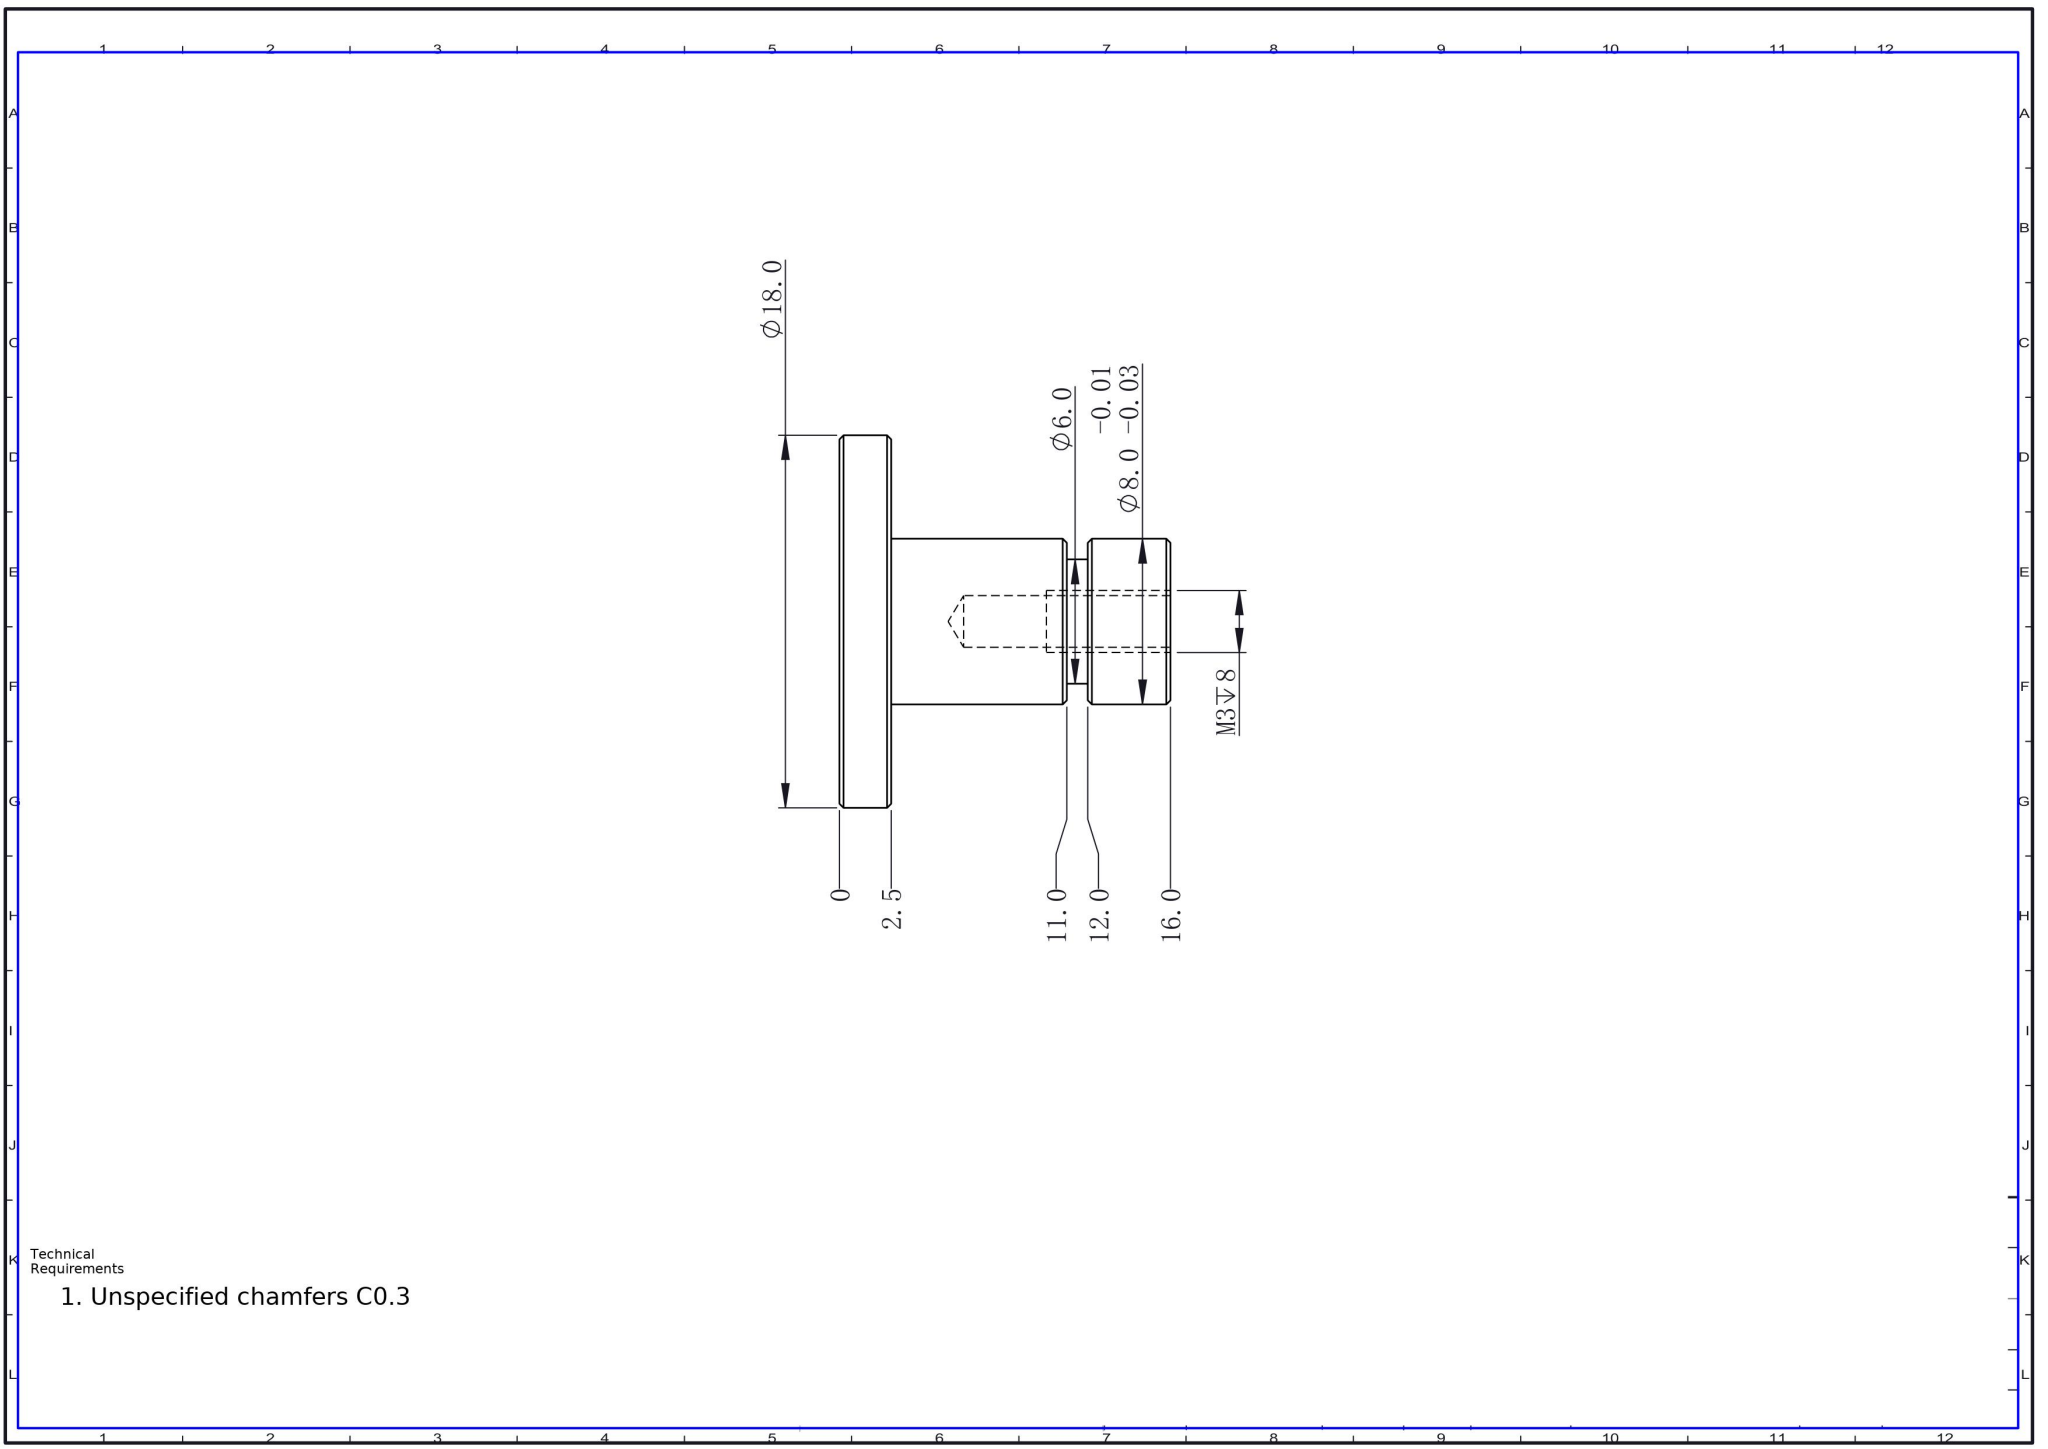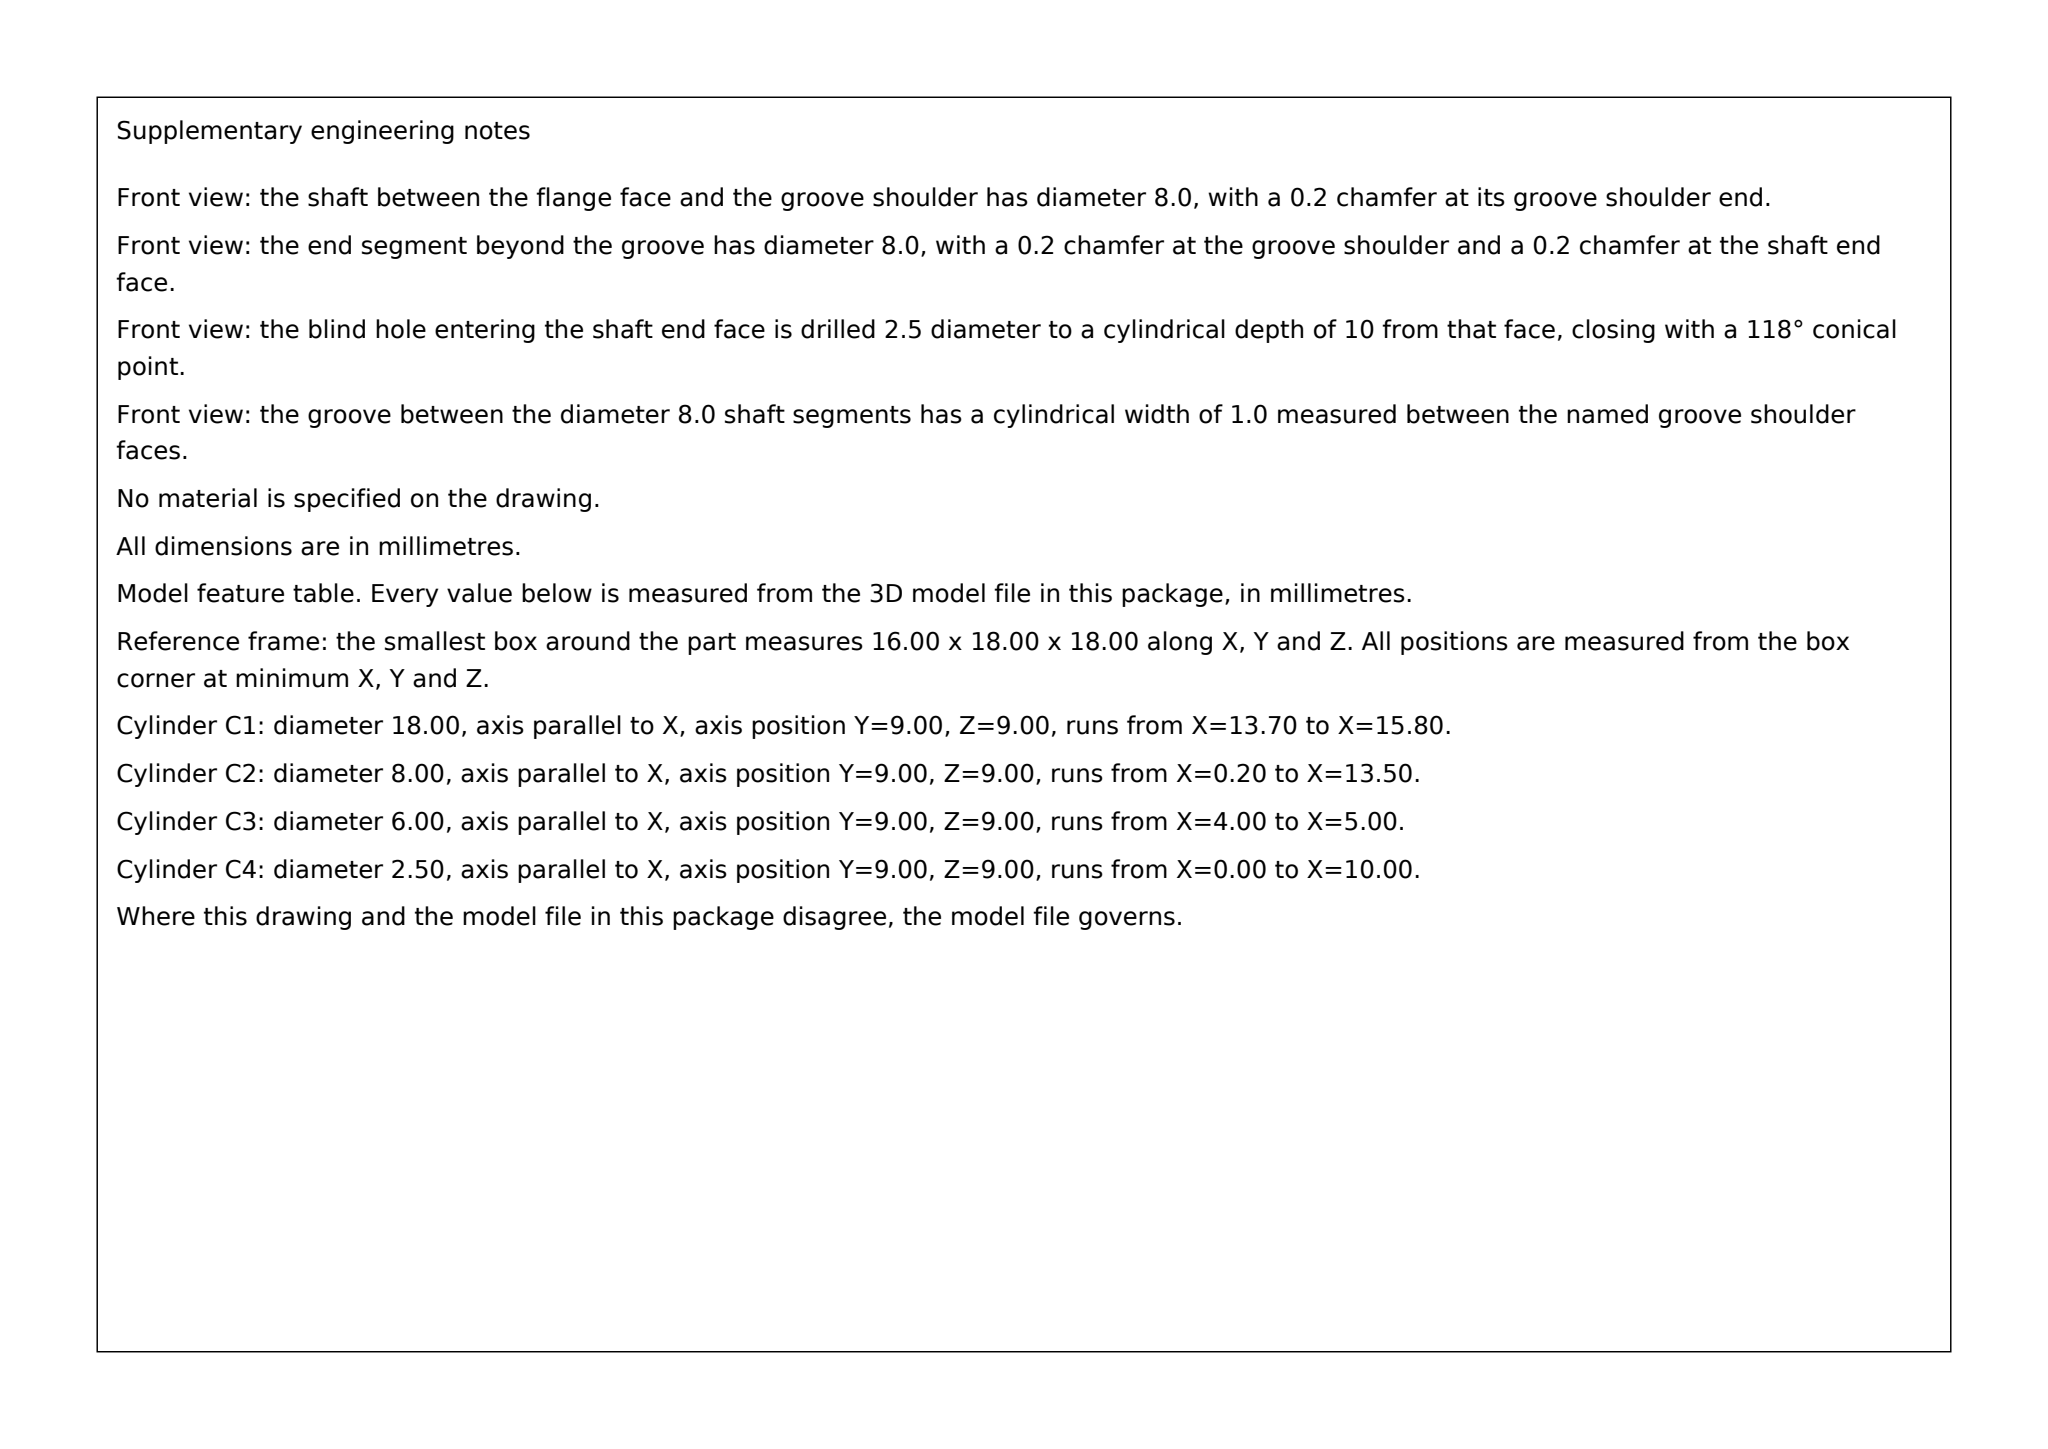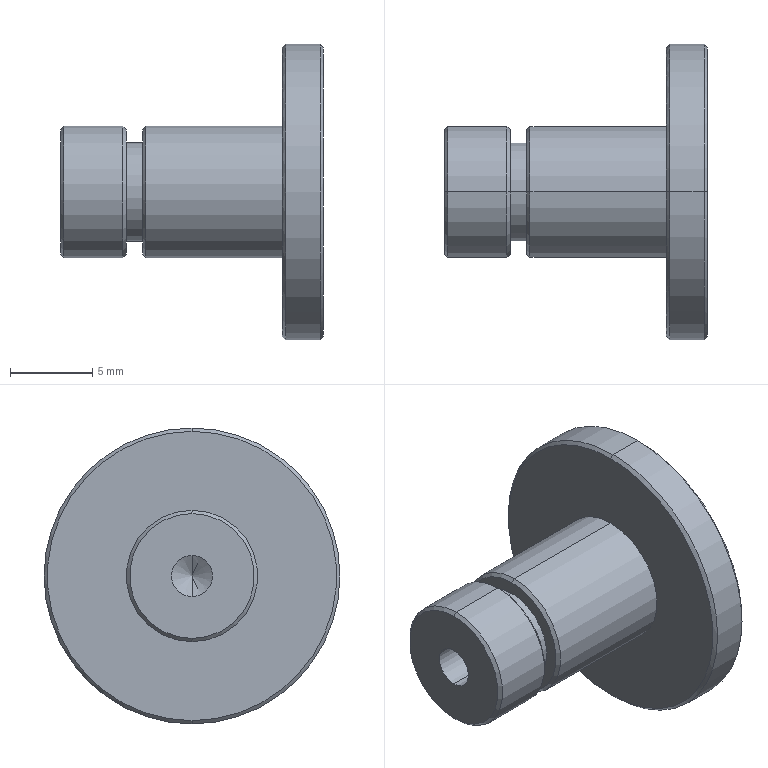Part | SolidWorks | mm | 1 solid | 27 faces | box 16 x 18 x 18 mm | volume 1239 mm3 | cone 12 | cylinder 10 | plane 5 | commonest cylinder face diameters 8 x4 2.5 x2 6 x2 18 x2
Drawing notes:
Ø8.0 SHAFT FROM FLANGE FACE (2.5) TO Ø6.0 GROOVE (11.0) | from the solid: cylinder dia 8.0, axis x, len 8.3 between 18.0 flange and 6.0 groove (2.5-11.0 nominal)
TAP DRILL Ø2.5 DP 10 FROM END FACE (16.0), 118° PT | from the solid: cylinder dia 2.5 axis x len 10.0 + cone 118° ref dia 2.5, open at x=16 end face
CHAMFER C0.2 x 45 ON BOTH Ø18 FLANGE OUTER EDGES (AT 0 AND 2.5 FROM FLANGE BACK FACE) | from the solid: cones[90.0,18.0] and cones[90.0,17.6]: (18.0-17.6)/2 = 0.2 chamfer leg at 45 deg on Ø18 cylinder (length 2.1, axis x)
CHAMFER C0.2 x 45 ON ALL Ø8 SHAFT AND BOSS END EDGES, INCL. END FACE AT 16.0 FROM FLANGE BACK FACE (0) | from the solid: cones[90.0,8.0] and cones[90.0,7.6] (4X): (8.0-7.6)/2 = 0.2 chamfer leg at 45 deg on Ø8 cylinders; x-planes at 13.5 and 16.0
STEP:
#1=CARTESIAN_POINT('',(9.,0.,-1.25));
#2=VERTEX_POINT('',#1);
#3=CARTESIAN_POINT('',(9.,0.,1.25));
#4=VERTEX_POINT('',#3);
#5=CARTESIAN_POINT('',(9.,0.,0.));
#6=DIRECTION('',(-1.,0.,0.));
#7=DIRECTION('',(0.,0.,1.));
#8=AXIS2_PLACEMENT_3D('',#5,#6,#7);
#9=CIRCLE('',#8,1.25);
#10=EDGE_CURVE('',#2,#4,#9,.T.);
#11=ORIENTED_EDGE('',*,*,#10,.F.);
#12=CARTESIAN_POINT('',(-1.,0.,-1.25));
#13=VERTEX_POINT('',#12);
#14=CARTESIAN_POINT('',(-1.,0.,-1.25));
#15=DIRECTION('',(-1.,0.,0.));
#16=VECTOR('',#15,1000.);
#17=LINE('',#14,#16);
#18=EDGE_CURVE('',#2,#13,#17,.T.);
#19=ORIENTED_EDGE('',*,*,#18,.T.);
#20=CARTESIAN_POINT('',(-1.,0.,1.25));
#21=VERTEX_POINT('',#20);
#22=CARTESIAN_POINT('',(-1.,0.,0.));
#23=DIRECTION('',(-1.,0.,0.));
#24=DIRECTION('',(0.,0.,1.));
#25=AXIS2_PLACEMENT_3D('',#22,#23,#24);
#26=CIRCLE('',#25,1.25);
#27=EDGE_CURVE('',#13,#21,#26,.T.);
#28=ORIENTED_EDGE('',*,*,#27,.T.);
#29=CARTESIAN_POINT('',(-1.,0.,1.25));
#30=DIRECTION('',(-1.,0.,0.));
#31=VECTOR('',#30,1000.);
#32=LINE('',#29,#31);
#33=EDGE_CURVE('',#4,#21,#32,.T.);
#34=ORIENTED_EDGE('',*,*,#33,.F.);
#35=EDGE_LOOP('',(#11,#19,#28,#34));
#36=FACE_OUTER_BOUND('',#35,.T.);
#37=CARTESIAN_POINT('',(-1.,0.,0.));
#38=DIRECTION('',(-1.,0.,0.));
#39=DIRECTION('',(0.,0.,1.));
#40=AXIS2_PLACEMENT_3D('',#37,#38,#39);
#41=CYLINDRICAL_SURFACE('',#40,1.25);
#42=ADVANCED_FACE('',(#36),#41,.F.);
#43=CARTESIAN_POINT('',(9.751,-0.,0.));
#44=VERTEX_POINT('',#43);
#45=CARTESIAN_POINT('',(9.,0.,1.25));
#46=DIRECTION('',(-0.515,0.,0.8572));
#47=VECTOR('',#46,1000.);
#48=LINE('',#45,#47);
#49=EDGE_CURVE('',#44,#4,#48,.T.);
#50=ORIENTED_EDGE('',*,*,#49,.F.);
#51=CARTESIAN_POINT('',(9.,0.,-1.25));
#52=DIRECTION('',(-0.515,0.,-0.8572));
#53=VECTOR('',#52,1000.);
#54=LINE('',#51,#53);
#55=EDGE_CURVE('',#44,#2,#54,.T.);
#56=ORIENTED_EDGE('',*,*,#55,.T.);
#57=ORIENTED_EDGE('',*,*,#10,.T.);
#58=EDGE_LOOP('',(#50,#56,#57));
#59=FACE_OUTER_BOUND('',#58,.T.);
#60=CARTESIAN_POINT('',(9.,0.,0.));
#61=DIRECTION('',(-1.,0.,0.));
#62=DIRECTION('',(0.,0.,1.));
#63=AXIS2_PLACEMENT_3D('',#60,#61,#62);
#64=CONICAL_SURFACE('',#63,1.25,1.03);
#65=ADVANCED_FACE('',(#59),#64,.F.);
#66=CARTESIAN_POINT('',(15.,0.,-8.8));
#67=VERTEX_POINT('',#66);
#68=CARTESIAN_POINT('',(15.,0.,8.8));
#69=VERTEX_POINT('',#68);
#70=CARTESIAN_POINT('',(15.,0.,0.));
#71=DIRECTION('',(1.,0.,0.));
#72=DIRECTION('',(0.,0.,1.));
#73=AXIS2_PLACEMENT_3D('',#70,#71,#72);
#74=CIRCLE('',#73,8.8);
#75=EDGE_CURVE('',#67,#69,#74,.T.);
#76=ORIENTED_EDGE('',*,*,#75,.F.);
#77=CARTESIAN_POINT('',(14.8,0.,-9.));
#78=VERTEX_POINT('',#77);
#79=CARTESIAN_POINT('',(14.8,0.,-9.));
#80=DIRECTION('',(-0.7071,0.,-0.7071));
#81=VECTOR('',#80,1000.);
#82=LINE('',#79,#81);
#83=EDGE_CURVE('',#67,#78,#82,.T.);
#84=ORIENTED_EDGE('',*,*,#83,.T.);
#85=CARTESIAN_POINT('',(14.8,0.,9.));
#86=VERTEX_POINT('',#85);
#87=CARTESIAN_POINT('',(14.8,0.,0.));
#88=DIRECTION('',(-1.,0.,0.));
#89=DIRECTION('',(0.,0.,1.));
#90=AXIS2_PLACEMENT_3D('',#87,#88,#89);
#91=CIRCLE('',#90,9.);
#92=EDGE_CURVE('',#86,#78,#91,.T.);
#93=ORIENTED_EDGE('',*,*,#92,.F.);
#94=CARTESIAN_POINT('',(14.8,0.,9.));
#95=DIRECTION('',(-0.7071,0.,0.7071));
#96=VECTOR('',#95,1000.);
#97=LINE('',#94,#96);
#98=EDGE_CURVE('',#69,#86,#97,.T.);
#99=ORIENTED_EDGE('',*,*,#98,.F.);
#100=EDGE_LOOP('',(#76,#84,#93,#99));
#101=FACE_OUTER_BOUND('',#100,.T.);
#102=CARTESIAN_POINT('',(14.8,0.,0.));
#103=DIRECTION('',(-1.,0.,0.));
#104=DIRECTION('',(0.,0.,1.));
#105=AXIS2_PLACEMENT_3D('',#102,#103,#104);
#106=CONICAL_SURFACE('',#105,9.,0.7854);
#107=ADVANCED_FACE('',(#101),#106,.T.);
#108=CARTESIAN_POINT('',(12.5,0.,8.8));
#109=VERTEX_POINT('',#108);
#110=CARTESIAN_POINT('',(12.5,0.,-8.8));
#111=VERTEX_POINT('',#110);
#112=CARTESIAN_POINT('',(12.5,0.,0.));
#113=DIRECTION('',(-1.,0.,0.));
#114=DIRECTION('',(0.,0.,-1.));
#115=AXIS2_PLACEMENT_3D('',#112,#113,#114);
#116=CIRCLE('',#115,8.8);
#117=EDGE_CURVE('',#109,#111,#116,.T.);
#118=ORIENTED_EDGE('',*,*,#117,.F.);
#119=CARTESIAN_POINT('',(12.7,0.,9.));
#120=VERTEX_POINT('',#119);
#121=CARTESIAN_POINT('',(12.5,0.,8.8));
#122=DIRECTION('',(0.7071,0.,0.7071));
#123=VECTOR('',#122,1000.);
#124=LINE('',#121,#123);
#125=EDGE_CURVE('',#109,#120,#124,.T.);
#126=ORIENTED_EDGE('',*,*,#125,.T.);
#127=CARTESIAN_POINT('',(12.7,0.,-9.));
#128=VERTEX_POINT('',#127);
#129=CARTESIAN_POINT('',(12.7,0.,0.));
#130=DIRECTION('',(1.,0.,0.));
#131=DIRECTION('',(0.,0.,-1.));
#132=AXIS2_PLACEMENT_3D('',#129,#130,#131);
#133=CIRCLE('',#132,9.);
#134=EDGE_CURVE('',#128,#120,#133,.T.);
#135=ORIENTED_EDGE('',*,*,#134,.F.);
#136=CARTESIAN_POINT('',(12.5,0.,-8.8));
#137=DIRECTION('',(0.7071,0.,-0.7071));
#138=VECTOR('',#137,1000.);
#139=LINE('',#136,#138);
#140=EDGE_CURVE('',#111,#128,#139,.T.);
#141=ORIENTED_EDGE('',*,*,#140,.F.);
#142=EDGE_LOOP('',(#118,#126,#135,#141));
#143=FACE_OUTER_BOUND('',#142,.T.);
#144=CARTESIAN_POINT('',(12.5,0.,0.));
#145=DIRECTION('',(1.,0.,0.));
#146=DIRECTION('',(0.,0.,-1.));
#147=AXIS2_PLACEMENT_3D('',#144,#145,#146);
#148=CONICAL_SURFACE('',#147,8.8,0.7854);
#149=ADVANCED_FACE('',(#143),#148,.T.);
#150=CARTESIAN_POINT('',(-1.,0.,3.8));
#151=VERTEX_POINT('',#150);
#152=CARTESIAN_POINT('',(-1.,0.,-3.8));
#153=VERTEX_POINT('',#152);
#154=CARTESIAN_POINT('',(-1.,0.,0.));
#155=DIRECTION('',(-1.,0.,0.));
#156=DIRECTION('',(0.,0.,-1.));
#157=AXIS2_PLACEMENT_3D('',#154,#155,#156);
#158=CIRCLE('',#157,3.8);
#159=EDGE_CURVE('',#151,#153,#158,.T.);
#160=ORIENTED_EDGE('',*,*,#159,.F.);
#161=CARTESIAN_POINT('',(-0.8,0.,4.));
#162=VERTEX_POINT('',#161);
#163=CARTESIAN_POINT('',(-1.,0.,3.8));
#164=DIRECTION('',(0.7071,0.,0.7071));
#165=VECTOR('',#164,1000.);
#166=LINE('',#163,#165);
#167=EDGE_CURVE('',#151,#162,#166,.T.);
#168=ORIENTED_EDGE('',*,*,#167,.T.);
#169=CARTESIAN_POINT('',(-0.8,0.,-4.));
#170=VERTEX_POINT('',#169);
#171=CARTESIAN_POINT('',(-0.8,0.,0.));
#172=DIRECTION('',(1.,0.,0.));
#173=DIRECTION('',(0.,0.,-1.));
#174=AXIS2_PLACEMENT_3D('',#171,#172,#173);
#175=CIRCLE('',#174,4.);
#176=EDGE_CURVE('',#170,#162,#175,.T.);
#177=ORIENTED_EDGE('',*,*,#176,.F.);
#178=CARTESIAN_POINT('',(-1.,0.,-3.8));
#179=DIRECTION('',(0.7071,0.,-0.7071));
#180=VECTOR('',#179,1000.);
#181=LINE('',#178,#180);
#182=EDGE_CURVE('',#153,#170,#181,.T.);
#183=ORIENTED_EDGE('',*,*,#182,.F.);
#184=EDGE_LOOP('',(#160,#168,#177,#183));
#185=FACE_OUTER_BOUND('',#184,.T.);
#186=CARTESIAN_POINT('',(-1.,0.,0.));
#187=DIRECTION('',(1.,0.,0.));
#188=DIRECTION('',(0.,0.,-1.));
#189=AXIS2_PLACEMENT_3D('',#186,#187,#188);
#190=CONICAL_SURFACE('',#189,3.8,0.7854);
#191=ADVANCED_FACE('',(#185),#190,.T.);
#192=CARTESIAN_POINT('',(4.,0.,3.8));
#193=VERTEX_POINT('',#192);
#194=CARTESIAN_POINT('',(4.,0.,-3.8));
#195=VERTEX_POINT('',#194);
#196=CARTESIAN_POINT('',(4.,0.,0.));
#197=DIRECTION('',(-1.,0.,0.));
#198=DIRECTION('',(0.,0.,1.));
#199=AXIS2_PLACEMENT_3D('',#196,#197,#198);
#200=CIRCLE('',#199,3.8);
#201=EDGE_CURVE('',#193,#195,#200,.T.);
#202=ORIENTED_EDGE('',*,*,#201,.F.);
#203=CARTESIAN_POINT('',(4.2,0.,4.));
#204=VERTEX_POINT('',#203);
#205=CARTESIAN_POINT('',(4.,0.,3.8));
#206=DIRECTION('',(0.7071,0.,0.7071));
#207=VECTOR('',#206,1000.);
#208=LINE('',#205,#207);
#209=EDGE_CURVE('',#193,#204,#208,.T.);
#210=ORIENTED_EDGE('',*,*,#209,.T.);
#211=CARTESIAN_POINT('',(4.2,0.,-4.));
#212=VERTEX_POINT('',#211);
#213=CARTESIAN_POINT('',(4.2,0.,0.));
#214=DIRECTION('',(1.,0.,0.));
#215=DIRECTION('',(0.,0.,1.));
#216=AXIS2_PLACEMENT_3D('',#213,#214,#215);
#217=CIRCLE('',#216,4.);
#218=EDGE_CURVE('',#212,#204,#217,.T.);
#219=ORIENTED_EDGE('',*,*,#218,.F.);
#220=CARTESIAN_POINT('',(4.,0.,-3.8));
#221=DIRECTION('',(0.7071,0.,-0.7071));
#222=VECTOR('',#221,1000.);
#223=LINE('',#220,#222);
#224=EDGE_CURVE('',#195,#212,#223,.T.);
#225=ORIENTED_EDGE('',*,*,#224,.F.);
#226=EDGE_LOOP('',(#202,#210,#219,#225));
#227=FACE_OUTER_BOUND('',#226,.T.);
#228=CARTESIAN_POINT('',(4.,0.,0.));
#229=DIRECTION('',(1.,0.,0.));
#230=DIRECTION('',(0.,0.,-1.));
#231=AXIS2_PLACEMENT_3D('',#228,#229,#230);
#232=CONICAL_SURFACE('',#231,3.8,0.7854);
#233=ADVANCED_FACE('',(#227),#232,.T.);
#234=CARTESIAN_POINT('',(3.,0.,-3.8));
#235=VERTEX_POINT('',#234);
#236=CARTESIAN_POINT('',(3.,0.,3.8));
#237=VERTEX_POINT('',#236);
#238=CARTESIAN_POINT('',(3.,0.,0.));
#239=DIRECTION('',(1.,0.,0.));
#240=DIRECTION('',(0.,0.,1.));
#241=AXIS2_PLACEMENT_3D('',#238,#239,#240);
#242=CIRCLE('',#241,3.8);
#243=EDGE_CURVE('',#235,#237,#242,.T.);
#244=ORIENTED_EDGE('',*,*,#243,.F.);
#245=CARTESIAN_POINT('',(2.8,0.,-4.));
#246=VERTEX_POINT('',#245);
#247=CARTESIAN_POINT('',(2.8,0.,-4.));
#248=DIRECTION('',(-0.7071,0.,-0.7071));
#249=VECTOR('',#248,1000.);
#250=LINE('',#247,#249);
#251=EDGE_CURVE('',#235,#246,#250,.T.);
#252=ORIENTED_EDGE('',*,*,#251,.T.);
#253=CARTESIAN_POINT('',(2.8,0.,4.));
#254=VERTEX_POINT('',#253);
#255=CARTESIAN_POINT('',(2.8,0.,0.));
#256=DIRECTION('',(-1.,0.,0.));
#257=DIRECTION('',(0.,0.,1.));
#258=AXIS2_PLACEMENT_3D('',#255,#256,#257);
#259=CIRCLE('',#258,4.);
#260=EDGE_CURVE('',#254,#246,#259,.T.);
#261=ORIENTED_EDGE('',*,*,#260,.F.);
#262=CARTESIAN_POINT('',(2.8,0.,4.));
#263=DIRECTION('',(-0.7071,0.,0.7071));
#264=VECTOR('',#263,1000.);
#265=LINE('',#262,#264);
#266=EDGE_CURVE('',#237,#254,#265,.T.);
#267=ORIENTED_EDGE('',*,*,#266,.F.);
#268=EDGE_LOOP('',(#244,#252,#261,#267));
#269=FACE_OUTER_BOUND('',#268,.T.);
#270=CARTESIAN_POINT('',(2.8,0.,0.));
#271=DIRECTION('',(-1.,0.,0.));
#272=DIRECTION('',(0.,0.,1.));
#273=AXIS2_PLACEMENT_3D('',#270,#271,#272);
#274=CONICAL_SURFACE('',#273,4.,0.7854);
#275=ADVANCED_FACE('',(#269),#274,.T.);
#276=ORIENTED_EDGE('',*,*,#260,.T.);
#277=CARTESIAN_POINT('',(0.,0.,-4.));
#278=DIRECTION('',(-1.,0.,0.));
#279=VECTOR('',#278,1000.);
#280=LINE('',#277,#279);
#281=EDGE_CURVE('',#246,#170,#280,.T.);
#282=ORIENTED_EDGE('',*,*,#281,.T.);
#283=ORIENTED_EDGE('',*,*,#176,.T.);
#284=CARTESIAN_POINT('',(0.,0.,4.));
#285=DIRECTION('',(-1.,0.,0.));
#286=VECTOR('',#285,1000.);
#287=LINE('',#284,#286);
#288=EDGE_CURVE('',#254,#162,#287,.T.);
#289=ORIENTED_EDGE('',*,*,#288,.F.);
#290=EDGE_LOOP('',(#276,#282,#283,#289));
#291=FACE_OUTER_BOUND('',#290,.T.);
#292=CARTESIAN_POINT('',(0.,0.,0.));
#293=DIRECTION('',(-1.,0.,0.));
#294=DIRECTION('',(0.,0.,1.));
#295=AXIS2_PLACEMENT_3D('',#292,#293,#294);
#296=CYLINDRICAL_SURFACE('',#295,4.);
#297=ADVANCED_FACE('',(#291),#296,.T.);
#298=CARTESIAN_POINT('',(3.,0.,3.));
#299=VERTEX_POINT('',#298);
#300=CARTESIAN_POINT('',(3.,0.,-3.));
#301=VERTEX_POINT('',#300);
#302=CARTESIAN_POINT('',(3.,0.,0.));
#303=DIRECTION('',(-1.,0.,0.));
#304=DIRECTION('',(0.,0.,1.));
#305=AXIS2_PLACEMENT_3D('',#302,#303,#304);
#306=CIRCLE('',#305,3.);
#307=EDGE_CURVE('',#299,#301,#306,.T.);
#308=ORIENTED_EDGE('',*,*,#307,.F.);
#309=CARTESIAN_POINT('',(4.,0.,3.));
#310=VERTEX_POINT('',#309);
#311=CARTESIAN_POINT('',(3.,0.,3.));
#312=DIRECTION('',(1.,0.,0.));
#313=VECTOR('',#312,1000.);
#314=LINE('',#311,#313);
#315=EDGE_CURVE('',#299,#310,#314,.T.);
#316=ORIENTED_EDGE('',*,*,#315,.T.);
#317=CARTESIAN_POINT('',(4.,0.,-3.));
#318=VERTEX_POINT('',#317);
#319=CARTESIAN_POINT('',(4.,0.,0.));
#320=DIRECTION('',(-1.,0.,0.));
#321=DIRECTION('',(0.,0.,1.));
#322=AXIS2_PLACEMENT_3D('',#319,#320,#321);
#323=CIRCLE('',#322,3.);
#324=EDGE_CURVE('',#310,#318,#323,.T.);
#325=ORIENTED_EDGE('',*,*,#324,.T.);
#326=CARTESIAN_POINT('',(3.,0.,-3.));
#327=DIRECTION('',(1.,0.,0.));
#328=VECTOR('',#327,1000.);
#329=LINE('',#326,#328);
#330=EDGE_CURVE('',#301,#318,#329,.T.);
#331=ORIENTED_EDGE('',*,*,#330,.F.);
#332=EDGE_LOOP('',(#308,#316,#325,#331));
#333=FACE_OUTER_BOUND('',#332,.T.);
#334=CARTESIAN_POINT('',(3.,0.,0.));
#335=DIRECTION('',(1.,0.,0.));
#336=DIRECTION('',(0.,0.,-1.));
#337=AXIS2_PLACEMENT_3D('',#334,#335,#336);
#338=CYLINDRICAL_SURFACE('',#337,3.);
#339=ADVANCED_FACE('',(#333),#338,.T.);
#340=ORIENTED_EDGE('',*,*,#92,.T.);
#341=CARTESIAN_POINT('',(-16.,0.,-9.));
#342=DIRECTION('',(-1.,0.,0.));
#343=VECTOR('',#342,1000.);
#344=LINE('',#341,#343);
#345=EDGE_CURVE('',#78,#128,#344,.T.);
#346=ORIENTED_EDGE('',*,*,#345,.T.);
#347=ORIENTED_EDGE('',*,*,#134,.T.);
#348=CARTESIAN_POINT('',(-16.,0.,9.));
#349=DIRECTION('',(-1.,0.,0.));
#350=VECTOR('',#349,1000.);
#351=LINE('',#348,#350);
#352=EDGE_CURVE('',#86,#120,#351,.T.);
#353=ORIENTED_EDGE('',*,*,#352,.F.);
#354=EDGE_LOOP('',(#340,#346,#347,#353));
#355=FACE_OUTER_BOUND('',#354,.T.);
#356=CARTESIAN_POINT('',(-16.,0.,0.));
#357=DIRECTION('',(-1.,0.,0.));
#358=DIRECTION('',(0.,0.,1.));
#359=AXIS2_PLACEMENT_3D('',#356,#357,#358);
#360=CYLINDRICAL_SURFACE('',#359,9.);
#361=ADVANCED_FACE('',(#355),#360,.T.);
#362=CARTESIAN_POINT('',(12.5,0.,4.));
#363=VERTEX_POINT('',#362);
#364=CARTESIAN_POINT('',(12.5,0.,-4.));
#365=VERTEX_POINT('',#364);
#366=CARTESIAN_POINT('',(12.5,0.,0.));
#367=DIRECTION('',(-1.,0.,0.));
#368=DIRECTION('',(0.,0.,1.));
#369=AXIS2_PLACEMENT_3D('',#366,#367,#368);
#370=CIRCLE('',#369,4.);
#371=EDGE_CURVE('',#363,#365,#370,.T.);
#372=ORIENTED_EDGE('',*,*,#371,.T.);
#373=CARTESIAN_POINT('',(0.,0.,-4.));
#374=DIRECTION('',(-1.,0.,0.));
#375=VECTOR('',#374,1000.);
#376=LINE('',#373,#375);
#377=EDGE_CURVE('',#365,#212,#376,.T.);
#378=ORIENTED_EDGE('',*,*,#377,.T.);
#379=ORIENTED_EDGE('',*,*,#218,.T.);
#380=CARTESIAN_POINT('',(0.,0.,4.));
#381=DIRECTION('',(-1.,0.,0.));
#382=VECTOR('',#381,1000.);
#383=LINE('',#380,#382);
#384=EDGE_CURVE('',#363,#204,#383,.T.);
#385=ORIENTED_EDGE('',*,*,#384,.F.);
#386=EDGE_LOOP('',(#372,#378,#379,#385));
#387=FACE_OUTER_BOUND('',#386,.T.);
#388=CARTESIAN_POINT('',(0.,0.,0.));
#389=DIRECTION('',(-1.,0.,0.));
#390=DIRECTION('',(0.,0.,1.));
#391=AXIS2_PLACEMENT_3D('',#388,#389,#390);
#392=CYLINDRICAL_SURFACE('',#391,4.);
#393=ADVANCED_FACE('',(#387),#392,.T.);
#394=ORIENTED_EDGE('',*,*,#377,.F.);
#395=CARTESIAN_POINT('',(12.5,0.,0.));
#396=DIRECTION('',(-1.,0.,0.));
#397=DIRECTION('',(0.,0.,1.));
#398=AXIS2_PLACEMENT_3D('',#395,#396,#397);
#399=CIRCLE('',#398,4.);
#400=EDGE_CURVE('',#365,#363,#399,.T.);
#401=ORIENTED_EDGE('',*,*,#400,.T.);
#402=ORIENTED_EDGE('',*,*,#384,.T.);
#403=CARTESIAN_POINT('',(4.2,0.,0.));
#404=DIRECTION('',(1.,0.,0.));
#405=DIRECTION('',(0.,0.,1.));
#406=AXIS2_PLACEMENT_3D('',#403,#404,#405);
#407=CIRCLE('',#406,4.);
#408=EDGE_CURVE('',#204,#212,#407,.T.);
#409=ORIENTED_EDGE('',*,*,#408,.T.);
#410=EDGE_LOOP('',(#394,#401,#402,#409));
#411=FACE_OUTER_BOUND('',#410,.T.);
#412=CARTESIAN_POINT('',(0.,0.,0.));
#413=DIRECTION('',(-1.,0.,0.));
#414=DIRECTION('',(0.,0.,1.));
#415=AXIS2_PLACEMENT_3D('',#412,#413,#414);
#416=CYLINDRICAL_SURFACE('',#415,4.);
#417=ADVANCED_FACE('',(#411),#416,.T.);
#418=CARTESIAN_POINT('',(12.5,0.,0.));
#419=DIRECTION('',(-1.,0.,0.));
#420=DIRECTION('',(0.,0.,-1.));
#421=AXIS2_PLACEMENT_3D('',#418,#419,#420);
#422=CIRCLE('',#421,8.8);
#423=EDGE_CURVE('',#111,#109,#422,.T.);
#424=ORIENTED_EDGE('',*,*,#423,.T.);
#425=ORIENTED_EDGE('',*,*,#117,.T.);
#426=EDGE_LOOP('',(#424,#425));
#427=FACE_OUTER_BOUND('',#426,.T.);
#428=ORIENTED_EDGE('',*,*,#371,.F.);
#429=ORIENTED_EDGE('',*,*,#400,.F.);
#430=EDGE_LOOP('',(#428,#429));
#431=FACE_BOUND('',#430,.T.);
#432=CARTESIAN_POINT('',(12.5,4.,0.));
#433=DIRECTION('',(1.,0.,0.));
#434=DIRECTION('',(0.,0.,-1.));
#435=AXIS2_PLACEMENT_3D('',#432,#433,#434);
#436=PLANE('',#435);
#437=ADVANCED_FACE('',(#427,#431),#436,.F.);
#438=ORIENTED_EDGE('',*,*,#345,.F.);
#439=CARTESIAN_POINT('',(14.8,0.,0.));
#440=DIRECTION('',(-1.,0.,0.));
#441=DIRECTION('',(0.,0.,1.));
#442=AXIS2_PLACEMENT_3D('',#439,#440,#441);
#443=CIRCLE('',#442,9.);
#444=EDGE_CURVE('',#78,#86,#443,.T.);
#445=ORIENTED_EDGE('',*,*,#444,.T.);
#446=ORIENTED_EDGE('',*,*,#352,.T.);
#447=CARTESIAN_POINT('',(12.7,0.,0.));
#448=DIRECTION('',(1.,0.,0.));
#449=DIRECTION('',(0.,0.,-1.));
#450=AXIS2_PLACEMENT_3D('',#447,#448,#449);
#451=CIRCLE('',#450,9.);
#452=EDGE_CURVE('',#120,#128,#451,.T.);
#453=ORIENTED_EDGE('',*,*,#452,.T.);
#454=EDGE_LOOP('',(#438,#445,#446,#453));
#455=FACE_OUTER_BOUND('',#454,.T.);
#456=CARTESIAN_POINT('',(-16.,0.,0.));
#457=DIRECTION('',(-1.,0.,0.));
#458=DIRECTION('',(0.,0.,1.));
#459=AXIS2_PLACEMENT_3D('',#456,#457,#458);
#460=CYLINDRICAL_SURFACE('',#459,9.);
#461=ADVANCED_FACE('',(#455),#460,.T.);
#462=CARTESIAN_POINT('',(15.,0.,0.));
#463=DIRECTION('',(1.,0.,0.));
#464=DIRECTION('',(0.,0.,1.));
#465=AXIS2_PLACEMENT_3D('',#462,#463,#464);
#466=CIRCLE('',#465,8.8);
#467=EDGE_CURVE('',#69,#67,#466,.T.);
#468=ORIENTED_EDGE('',*,*,#467,.T.);
#469=ORIENTED_EDGE('',*,*,#75,.T.);
#470=EDGE_LOOP('',(#468,#469));
#471=FACE_OUTER_BOUND('',#470,.T.);
#472=CARTESIAN_POINT('',(15.,9.,0.));
#473=DIRECTION('',(-1.,0.,0.));
#474=DIRECTION('',(0.,0.,1.));
#475=AXIS2_PLACEMENT_3D('',#472,#473,#474);
#476=PLANE('',#475);
#477=ADVANCED_FACE('',(#471),#476,.F.);
#478=CARTESIAN_POINT('',(3.,0.,0.));
#479=DIRECTION('',(1.,0.,0.));
#480=DIRECTION('',(0.,0.,1.));
#481=AXIS2_PLACEMENT_3D('',#478,#479,#480);
#482=CIRCLE('',#481,3.8);
#483=EDGE_CURVE('',#237,#235,#482,.T.);
#484=ORIENTED_EDGE('',*,*,#483,.T.);
#485=ORIENTED_EDGE('',*,*,#243,.T.);
#486=EDGE_LOOP('',(#484,#485));
#487=FACE_OUTER_BOUND('',#486,.T.);
#488=CARTESIAN_POINT('',(3.,0.,0.));
#489=DIRECTION('',(-1.,0.,0.));
#490=DIRECTION('',(0.,0.,1.));
#491=AXIS2_PLACEMENT_3D('',#488,#489,#490);
#492=CIRCLE('',#491,3.);
#493=EDGE_CURVE('',#301,#299,#492,.T.);
#494=ORIENTED_EDGE('',*,*,#493,.T.);
#495=ORIENTED_EDGE('',*,*,#307,.T.);
#496=EDGE_LOOP('',(#494,#495));
#497=FACE_BOUND('',#496,.T.);
#498=CARTESIAN_POINT('',(3.,0.,0.));
#499=DIRECTION('',(-1.,0.,0.));
#500=DIRECTION('',(0.,0.,1.));
#501=AXIS2_PLACEMENT_3D('',#498,#499,#500);
#502=PLANE('',#501);
#503=ADVANCED_FACE('',(#487,#497),#502,.F.);
#504=CARTESIAN_POINT('',(4.,0.,0.));
#505=DIRECTION('',(-1.,0.,0.));
#506=DIRECTION('',(0.,0.,1.));
#507=AXIS2_PLACEMENT_3D('',#504,#505,#506);
#508=CIRCLE('',#507,3.8);
#509=EDGE_CURVE('',#195,#193,#508,.T.);
#510=ORIENTED_EDGE('',*,*,#509,.T.);
#511=ORIENTED_EDGE('',*,*,#201,.T.);
#512=EDGE_LOOP('',(#510,#511));
#513=FACE_OUTER_BOUND('',#512,.T.);
#514=CARTESIAN_POINT('',(4.,0.,0.));
#515=DIRECTION('',(-1.,0.,0.));
#516=DIRECTION('',(0.,0.,1.));
#517=AXIS2_PLACEMENT_3D('',#514,#515,#516);
#518=CIRCLE('',#517,3.);
#519=EDGE_CURVE('',#318,#310,#518,.T.);
#520=ORIENTED_EDGE('',*,*,#519,.F.);
#521=ORIENTED_EDGE('',*,*,#324,.F.);
#522=EDGE_LOOP('',(#520,#521));
#523=FACE_BOUND('',#522,.T.);
#524=CARTESIAN_POINT('',(4.,0.,0.));
#525=DIRECTION('',(-1.,0.,0.));
#526=DIRECTION('',(0.,0.,1.));
#527=AXIS2_PLACEMENT_3D('',#524,#525,#526);
#528=PLANE('',#527);
#529=ADVANCED_FACE('',(#513,#523),#528,.T.);
#530=ORIENTED_EDGE('',*,*,#315,.F.);
#531=ORIENTED_EDGE('',*,*,#493,.F.);
#532=ORIENTED_EDGE('',*,*,#330,.T.);
#533=ORIENTED_EDGE('',*,*,#519,.T.);
#534=EDGE_LOOP('',(#530,#531,#532,#533));
#535=FACE_OUTER_BOUND('',#534,.T.);
#536=CARTESIAN_POINT('',(3.,0.,0.));
#537=DIRECTION('',(1.,0.,0.));
#538=DIRECTION('',(0.,0.,-1.));
#539=AXIS2_PLACEMENT_3D('',#536,#537,#538);
#540=CYLINDRICAL_SURFACE('',#539,3.);
#541=ADVANCED_FACE('',(#535),#540,.T.);
#542=CARTESIAN_POINT('',(-1.,0.,0.));
#543=DIRECTION('',(-1.,0.,0.));
#544=DIRECTION('',(0.,0.,1.));
#545=AXIS2_PLACEMENT_3D('',#542,#543,#544);
#546=CIRCLE('',#545,1.25);
#547=EDGE_CURVE('',#21,#13,#546,.T.);
#548=ORIENTED_EDGE('',*,*,#547,.F.);
#549=ORIENTED_EDGE('',*,*,#27,.F.);
#550=EDGE_LOOP('',(#548,#549));
#551=FACE_BOUND('',#550,.T.);
#552=CARTESIAN_POINT('',(-1.,0.,0.));
#553=DIRECTION('',(-1.,0.,0.));
#554=DIRECTION('',(0.,0.,-1.));
#555=AXIS2_PLACEMENT_3D('',#552,#553,#554);
#556=CIRCLE('',#555,3.8);
#557=EDGE_CURVE('',#153,#151,#556,.T.);
#558=ORIENTED_EDGE('',*,*,#557,.T.);
#559=ORIENTED_EDGE('',*,*,#159,.T.);
#560=EDGE_LOOP('',(#558,#559));
#561=FACE_OUTER_BOUND('',#560,.T.);
#562=CARTESIAN_POINT('',(-1.,0.,0.));
#563=DIRECTION('',(1.,0.,0.));
#564=DIRECTION('',(0.,0.,-1.));
#565=AXIS2_PLACEMENT_3D('',#562,#563,#564);
#566=PLANE('',#565);
#567=ADVANCED_FACE('',(#551,#561),#566,.F.);
#568=ORIENTED_EDGE('',*,*,#281,.F.);
#569=CARTESIAN_POINT('',(2.8,0.,0.));
#570=DIRECTION('',(-1.,0.,0.));
#571=DIRECTION('',(0.,0.,1.));
#572=AXIS2_PLACEMENT_3D('',#569,#570,#571);
#573=CIRCLE('',#572,4.);
#574=EDGE_CURVE('',#246,#254,#573,.T.);
#575=ORIENTED_EDGE('',*,*,#574,.T.);
#576=ORIENTED_EDGE('',*,*,#288,.T.);
#577=CARTESIAN_POINT('',(-0.8,0.,0.));
#578=DIRECTION('',(1.,0.,0.));
#579=DIRECTION('',(0.,0.,-1.));
#580=AXIS2_PLACEMENT_3D('',#577,#578,#579);
#581=CIRCLE('',#580,4.);
#582=EDGE_CURVE('',#162,#170,#581,.T.);
#583=ORIENTED_EDGE('',*,*,#582,.T.);
#584=EDGE_LOOP('',(#568,#575,#576,#583));
#585=FACE_OUTER_BOUND('',#584,.T.);
#586=CARTESIAN_POINT('',(0.,0.,0.));
#587=DIRECTION('',(-1.,0.,0.));
#588=DIRECTION('',(0.,0.,1.));
#589=AXIS2_PLACEMENT_3D('',#586,#587,#588);
#590=CYLINDRICAL_SURFACE('',#589,4.);
#591=ADVANCED_FACE('',(#585),#590,.T.);
#592=ORIENTED_EDGE('',*,*,#251,.F.);
#593=ORIENTED_EDGE('',*,*,#483,.F.);
#594=ORIENTED_EDGE('',*,*,#266,.T.);
#595=ORIENTED_EDGE('',*,*,#574,.F.);
#596=EDGE_LOOP('',(#592,#593,#594,#595));
#597=FACE_OUTER_BOUND('',#596,.T.);
#598=CARTESIAN_POINT('',(2.8,0.,0.));
#599=DIRECTION('',(-1.,0.,0.));
#600=DIRECTION('',(0.,0.,1.));
#601=AXIS2_PLACEMENT_3D('',#598,#599,#600);
#602=CONICAL_SURFACE('',#601,4.,0.7854);
#603=ADVANCED_FACE('',(#597),#602,.T.);
#604=ORIENTED_EDGE('',*,*,#209,.F.);
#605=ORIENTED_EDGE('',*,*,#509,.F.);
#606=ORIENTED_EDGE('',*,*,#224,.T.);
#607=ORIENTED_EDGE('',*,*,#408,.F.);
#608=EDGE_LOOP('',(#604,#605,#606,#607));
#609=FACE_OUTER_BOUND('',#608,.T.);
#610=CARTESIAN_POINT('',(4.,0.,0.));
#611=DIRECTION('',(1.,0.,0.));
#612=DIRECTION('',(0.,0.,-1.));
#613=AXIS2_PLACEMENT_3D('',#610,#611,#612);
#614=CONICAL_SURFACE('',#613,3.8,0.7854);
#615=ADVANCED_FACE('',(#609),#614,.T.);
#616=ORIENTED_EDGE('',*,*,#167,.F.);
#617=ORIENTED_EDGE('',*,*,#557,.F.);
#618=ORIENTED_EDGE('',*,*,#182,.T.);
#619=ORIENTED_EDGE('',*,*,#582,.F.);
#620=EDGE_LOOP('',(#616,#617,#618,#619));
#621=FACE_OUTER_BOUND('',#620,.T.);
#622=CARTESIAN_POINT('',(-1.,0.,0.));
#623=DIRECTION('',(1.,0.,0.));
#624=DIRECTION('',(0.,0.,-1.));
#625=AXIS2_PLACEMENT_3D('',#622,#623,#624);
#626=CONICAL_SURFACE('',#625,3.8,0.7854);
#627=ADVANCED_FACE('',(#621),#626,.T.);
#628=ORIENTED_EDGE('',*,*,#125,.F.);
#629=ORIENTED_EDGE('',*,*,#423,.F.);
#630=ORIENTED_EDGE('',*,*,#140,.T.);
#631=ORIENTED_EDGE('',*,*,#452,.F.);
#632=EDGE_LOOP('',(#628,#629,#630,#631));
#633=FACE_OUTER_BOUND('',#632,.T.);
#634=CARTESIAN_POINT('',(12.5,0.,0.));
#635=DIRECTION('',(1.,0.,0.));
#636=DIRECTION('',(0.,0.,-1.));
#637=AXIS2_PLACEMENT_3D('',#634,#635,#636);
#638=CONICAL_SURFACE('',#637,8.8,0.7854);
#639=ADVANCED_FACE('',(#633),#638,.T.);
#640=ORIENTED_EDGE('',*,*,#83,.F.);
#641=ORIENTED_EDGE('',*,*,#467,.F.);
#642=ORIENTED_EDGE('',*,*,#98,.T.);
#643=ORIENTED_EDGE('',*,*,#444,.F.);
#644=EDGE_LOOP('',(#640,#641,#642,#643));
#645=FACE_OUTER_BOUND('',#644,.T.);
#646=CARTESIAN_POINT('',(14.8,0.,0.));
#647=DIRECTION('',(-1.,0.,0.));
#648=DIRECTION('',(0.,0.,1.));
#649=AXIS2_PLACEMENT_3D('',#646,#647,#648);
#650=CONICAL_SURFACE('',#649,9.,0.7854);
#651=ADVANCED_FACE('',(#645),#650,.T.);
#652=ORIENTED_EDGE('',*,*,#55,.F.);
#653=ORIENTED_EDGE('',*,*,#49,.T.);
#654=CARTESIAN_POINT('',(9.,0.,0.));
#655=DIRECTION('',(-1.,0.,0.));
#656=DIRECTION('',(0.,0.,1.));
#657=AXIS2_PLACEMENT_3D('',#654,#655,#656);
#658=CIRCLE('',#657,1.25);
#659=EDGE_CURVE('',#4,#2,#658,.T.);
#660=ORIENTED_EDGE('',*,*,#659,.T.);
#661=EDGE_LOOP('',(#652,#653,#660));
#662=FACE_OUTER_BOUND('',#661,.T.);
#663=CARTESIAN_POINT('',(9.,0.,0.));
#664=DIRECTION('',(-1.,0.,0.));
#665=DIRECTION('',(0.,0.,1.));
#666=AXIS2_PLACEMENT_3D('',#663,#664,#665);
#667=CONICAL_SURFACE('',#666,1.25,1.03);
#668=ADVANCED_FACE('',(#662),#667,.F.);
#669=ORIENTED_EDGE('',*,*,#18,.F.);
#670=ORIENTED_EDGE('',*,*,#659,.F.);
#671=ORIENTED_EDGE('',*,*,#33,.T.);
#672=ORIENTED_EDGE('',*,*,#547,.T.);
#673=EDGE_LOOP('',(#669,#670,#671,#672));
#674=FACE_OUTER_BOUND('',#673,.T.);
#675=CARTESIAN_POINT('',(-1.,0.,0.));
#676=DIRECTION('',(-1.,0.,0.));
#677=DIRECTION('',(0.,0.,1.));
#678=AXIS2_PLACEMENT_3D('',#675,#676,#677);
#679=CYLINDRICAL_SURFACE('',#678,1.25);
#680=ADVANCED_FACE('',(#674),#679,.F.);
#681=CLOSED_SHELL('',(#42,#65,#107,#149,#191,#233,#275,#297,#339,#361,#393,#417,#437,#461,#477,#503,#529,#541,#567,#591,#603,#615,#627,#639,#651,#668,#680));
#682=MANIFOLD_SOLID_BREP('',#681);
#683=CARTESIAN_POINT('',(0.,0.,0.));
#684=DIRECTION('',(0.,0.,1.));
#685=DIRECTION('',(1.,0.,0.));
#686=AXIS2_PLACEMENT_3D('',#683,#684,#685);
#687=(LENGTH_UNIT()NAMED_UNIT(*)SI_UNIT(.MILLI.,.METRE.));
#688=UNCERTAINTY_MEASURE_WITH_UNIT(LENGTH_MEASURE(0.00001),#687,'','');
#689=(NAMED_UNIT(*)PLANE_ANGLE_UNIT()SI_UNIT($,.RADIAN.));
#690=(NAMED_UNIT(*)SI_UNIT($,.STERADIAN.)SOLID_ANGLE_UNIT());
#691=(GEOMETRIC_REPRESENTATION_CONTEXT(3)GLOBAL_UNCERTAINTY_ASSIGNED_CONTEXT((#688))GLOBAL_UNIT_ASSIGNED_CONTEXT((#687,#689,#690))REPRESENTATION_CONTEXT('',''));
#692=ADVANCED_BREP_SHAPE_REPRESENTATION('',(#682,#686),#691);